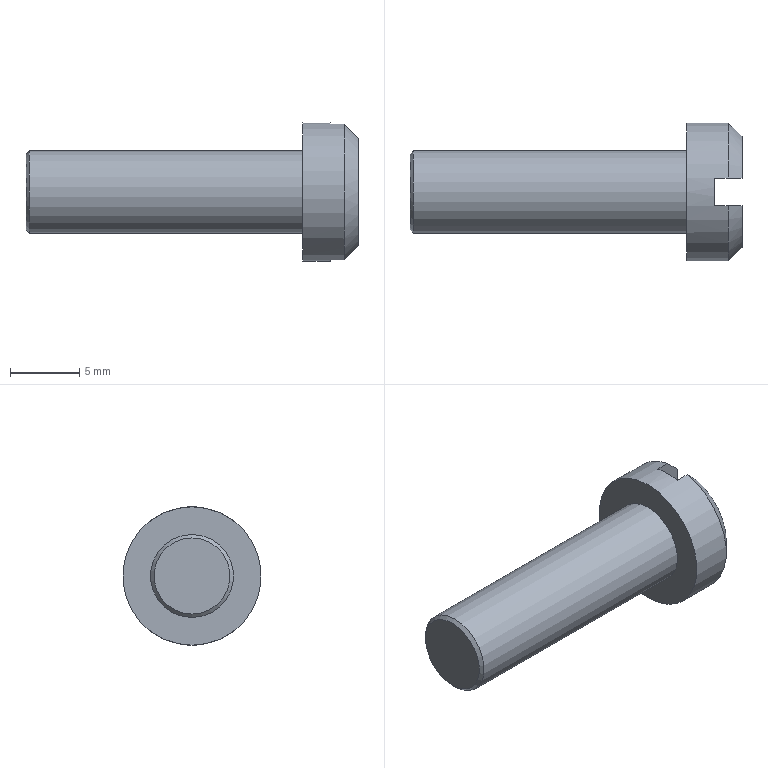Component | NX | SCREW2_2 | 1 solid | 12 faces | box 24 x 10 x 10 mm | volume 827 mm3 | plane 7 | cone 3 | cylinder 2 | commonest cylinder face diameters 10 x1 6 x1
STEP:
#1=CARTESIAN_POINT('',(0.,0.,0.));
#2=DIRECTION('',(0.,0.,1.));
#3=DIRECTION('',(1.,0.,0.));
#4=AXIS2_PLACEMENT_3D('',#1,#2,#3);
#5=CARTESIAN_POINT('',(54.,39.,45.627));
#6=VERTEX_POINT('',#5);
#7=CARTESIAN_POINT('',(54.,39.,53.373));
#8=VERTEX_POINT('',#7);
#9=CARTESIAN_POINT('',(54.,39.,42.282));
#10=DIRECTION('',(0.,0.,1.));
#11=VECTOR('',#10,1.);
#12=LINE('',#9,#11);
#13=CARTESIAN_POINT('',(54.,40.,49.5));
#14=DIRECTION('',(1.,0.,0.));
#15=DIRECTION('',(0.,0.,-1.));
#16=AXIS2_PLACEMENT_3D('',#13,#14,#15);
#17=PLANE('',#16);
#18=CARTESIAN_POINT('',(7.218,-1.));
#19=DIRECTION('',(-1.,0.));
#20=VECTOR('',#19,1.);
#21=LINE('',#18,#20);
#22=(GEOMETRIC_REPRESENTATION_CONTEXT(2)PARAMETRIC_REPRESENTATION_CONTEXT()REPRESENTATION_CONTEXT('',''));
#23=DEFINITIONAL_REPRESENTATION('',(#21),#22);
#24=PCURVE('',#17,#23);
#25=CARTESIAN_POINT('',(52.,39.,42.282));
#26=DIRECTION('',(0.,1.,0.));
#27=DIRECTION('',(1.,0.,0.));
#28=AXIS2_PLACEMENT_3D('',#25,#26,#27);
#29=PLANE('',#28);
#30=CARTESIAN_POINT('',(2.,0.));
#31=DIRECTION('',(0.,-1.));
#32=VECTOR('',#31,1.);
#33=LINE('',#30,#32);
#34=(GEOMETRIC_REPRESENTATION_CONTEXT(2)PARAMETRIC_REPRESENTATION_CONTEXT()REPRESENTATION_CONTEXT('',''));
#35=DEFINITIONAL_REPRESENTATION('',(#33),#34);
#36=PCURVE('',#29,#35);
#37=SURFACE_CURVE('',#12,(#24,#36),.PCURVE_S1.);
#38=EDGE_CURVE('',#6,#8,#37,.T.);
#39=ORIENTED_EDGE('',*,*,#38,.T.);
#40=CARTESIAN_POINT('',(54.,40.,49.5));
#41=DIRECTION('',(1.,0.,0.));
#42=DIRECTION('',(0.,0.,-1.));
#43=AXIS2_PLACEMENT_3D('',#40,#41,#42);
#44=CIRCLE('',#43,4.);
#45=CARTESIAN_POINT('',(0.,0.));
#46=DIRECTION('',(1.,0.));
#47=AXIS2_PLACEMENT_2D('',#45,#46);
#48=CIRCLE('',#47,4.);
#49=(GEOMETRIC_REPRESENTATION_CONTEXT(2)PARAMETRIC_REPRESENTATION_CONTEXT()REPRESENTATION_CONTEXT('',''));
#50=DEFINITIONAL_REPRESENTATION('',(#48),#49);
#51=PCURVE('',#17,#50);
#52=CARTESIAN_POINT('',(54.,40.,49.5));
#53=DIRECTION('',(-1.,0.,0.));
#54=DIRECTION('',(0.,0.,1.));
#55=AXIS2_PLACEMENT_3D('',#52,#53,#54);
#56=CONICAL_SURFACE('',#55,4.,0.7854);
#57=CARTESIAN_POINT('',(9.425,0.));
#58=DIRECTION('',(-1.,-0.));
#59=VECTOR('',#58,1.);
#60=LINE('',#57,#59);
#61=(GEOMETRIC_REPRESENTATION_CONTEXT(2)PARAMETRIC_REPRESENTATION_CONTEXT()REPRESENTATION_CONTEXT('',''));
#62=DEFINITIONAL_REPRESENTATION('',(#60),#61);
#63=PCURVE('',#56,#62);
#64=SURFACE_CURVE('',#44,(#51,#63),.PCURVE_S1.);
#65=EDGE_CURVE('',#8,#6,#64,.T.);
#66=ORIENTED_EDGE('',*,*,#65,.T.);
#67=EDGE_LOOP('',(#39,#66));
#68=FACE_BOUND('',#67,.T.);
#69=ADVANCED_FACE('',(#68),#17,.T.);
#70=CARTESIAN_POINT('',(54.,41.,53.373));
#71=VERTEX_POINT('',#70);
#72=CARTESIAN_POINT('',(54.,41.,45.627));
#73=VERTEX_POINT('',#72);
#74=CARTESIAN_POINT('',(54.,41.,56.718));
#75=DIRECTION('',(0.,0.,-1.));
#76=VECTOR('',#75,1.);
#77=LINE('',#74,#76);
#78=CARTESIAN_POINT('',(54.,40.,49.5));
#79=DIRECTION('',(1.,0.,0.));
#80=DIRECTION('',(0.,0.,-1.));
#81=AXIS2_PLACEMENT_3D('',#78,#79,#80);
#82=PLANE('',#81);
#83=CARTESIAN_POINT('',(-7.218,1.));
#84=DIRECTION('',(1.,0.));
#85=VECTOR('',#84,1.);
#86=LINE('',#83,#85);
#87=(GEOMETRIC_REPRESENTATION_CONTEXT(2)PARAMETRIC_REPRESENTATION_CONTEXT()REPRESENTATION_CONTEXT('',''));
#88=DEFINITIONAL_REPRESENTATION('',(#86),#87);
#89=PCURVE('',#82,#88);
#90=CARTESIAN_POINT('',(52.,41.,56.718));
#91=DIRECTION('',(0.,-1.,0.));
#92=DIRECTION('',(-1.,0.,0.));
#93=AXIS2_PLACEMENT_3D('',#90,#91,#92);
#94=PLANE('',#93);
#95=CARTESIAN_POINT('',(-2.,0.));
#96=DIRECTION('',(0.,1.));
#97=VECTOR('',#96,1.);
#98=LINE('',#95,#97);
#99=(GEOMETRIC_REPRESENTATION_CONTEXT(2)PARAMETRIC_REPRESENTATION_CONTEXT()REPRESENTATION_CONTEXT('',''));
#100=DEFINITIONAL_REPRESENTATION('',(#98),#99);
#101=PCURVE('',#94,#100);
#102=SURFACE_CURVE('',#77,(#89,#101),.PCURVE_S1.);
#103=EDGE_CURVE('',#71,#73,#102,.T.);
#104=ORIENTED_EDGE('',*,*,#103,.T.);
#105=CARTESIAN_POINT('',(54.,40.,49.5));
#106=DIRECTION('',(1.,0.,0.));
#107=DIRECTION('',(0.,0.,-1.));
#108=AXIS2_PLACEMENT_3D('',#105,#106,#107);
#109=CIRCLE('',#108,4.);
#110=CARTESIAN_POINT('',(0.,0.));
#111=DIRECTION('',(1.,0.));
#112=AXIS2_PLACEMENT_2D('',#110,#111);
#113=CIRCLE('',#112,4.);
#114=(GEOMETRIC_REPRESENTATION_CONTEXT(2)PARAMETRIC_REPRESENTATION_CONTEXT()REPRESENTATION_CONTEXT('',''));
#115=DEFINITIONAL_REPRESENTATION('',(#113),#114);
#116=PCURVE('',#82,#115);
#117=CARTESIAN_POINT('',(54.,40.,49.5));
#118=DIRECTION('',(-1.,0.,0.));
#119=DIRECTION('',(0.,0.,1.));
#120=AXIS2_PLACEMENT_3D('',#117,#118,#119);
#121=CONICAL_SURFACE('',#120,4.,0.7854);
#122=CARTESIAN_POINT('',(3.142,0.));
#123=DIRECTION('',(-1.,0.));
#124=VECTOR('',#123,1.);
#125=LINE('',#122,#124);
#126=(GEOMETRIC_REPRESENTATION_CONTEXT(2)PARAMETRIC_REPRESENTATION_CONTEXT()REPRESENTATION_CONTEXT('',''));
#127=DEFINITIONAL_REPRESENTATION('',(#125),#126);
#128=PCURVE('',#121,#127);
#129=SURFACE_CURVE('',#109,(#116,#128),.PCURVE_S1.);
#130=EDGE_CURVE('',#73,#71,#129,.T.);
#131=ORIENTED_EDGE('',*,*,#130,.T.);
#132=EDGE_LOOP('',(#104,#131));
#133=FACE_BOUND('',#132,.T.);
#134=ADVANCED_FACE('',(#133),#82,.T.);
#135=CARTESIAN_POINT('',(50.,40.,44.5));
#136=VERTEX_POINT('',#135);
#137=CARTESIAN_POINT('',(50.,40.,49.5));
#138=DIRECTION('',(1.,0.,0.));
#139=DIRECTION('',(0.,0.,-1.));
#140=AXIS2_PLACEMENT_3D('',#137,#138,#139);
#141=CIRCLE('',#140,5.);
#142=CARTESIAN_POINT('',(50.,40.,49.5));
#143=DIRECTION('',(1.,0.,0.));
#144=DIRECTION('',(0.,0.,-1.));
#145=AXIS2_PLACEMENT_3D('',#142,#143,#144);
#146=CYLINDRICAL_SURFACE('',#145,5.);
#147=CARTESIAN_POINT('',(0.,0.));
#148=DIRECTION('',(1.,0.));
#149=VECTOR('',#148,1.);
#150=LINE('',#147,#149);
#151=(GEOMETRIC_REPRESENTATION_CONTEXT(2)PARAMETRIC_REPRESENTATION_CONTEXT()REPRESENTATION_CONTEXT('',''));
#152=DEFINITIONAL_REPRESENTATION('',(#150),#151);
#153=PCURVE('',#146,#152);
#154=CARTESIAN_POINT('',(50.,40.,49.5));
#155=DIRECTION('',(-1.,0.,0.));
#156=DIRECTION('',(0.,0.,1.));
#157=AXIS2_PLACEMENT_3D('',#154,#155,#156);
#158=PLANE('',#157);
#159=CARTESIAN_POINT('',(-5.,0.));
#160=CARTESIAN_POINT('',(-5.,8.66));
#161=CARTESIAN_POINT('',(2.5,4.33));
#162=CARTESIAN_POINT('',(10.,0.));
#163=CARTESIAN_POINT('',(2.5,-4.33));
#164=CARTESIAN_POINT('',(-5.,-8.66));
#165=CARTESIAN_POINT('',(-5.,0.));
#166=(BOUNDED_CURVE()B_SPLINE_CURVE(2,(#159,#160,#161,#162,#163,#164,#165),.UNSPECIFIED.,.T.,.F.)B_SPLINE_CURVE_WITH_KNOTS((1,2,2,2,2,1),(-2.094,0.,2.094,4.189,6.283,8.378),.UNSPECIFIED.)CURVE()GEOMETRIC_REPRESENTATION_ITEM()RATIONAL_B_SPLINE_CURVE((1.,0.5,1.,0.5,1.,0.5,1.))REPRESENTATION_ITEM(''));
#167=(GEOMETRIC_REPRESENTATION_CONTEXT(2)PARAMETRIC_REPRESENTATION_CONTEXT()REPRESENTATION_CONTEXT('',''));
#168=DEFINITIONAL_REPRESENTATION('',(#166),#167);
#169=PCURVE('',#158,#168);
#170=SURFACE_CURVE('',#141,(#153,#169),.PCURVE_S1.);
#171=EDGE_CURVE('',#136,#136,#170,.T.);
#172=ORIENTED_EDGE('',*,*,#171,.T.);
#173=CARTESIAN_POINT('',(52.,40.,44.5));
#174=VERTEX_POINT('',#173);
#175=CARTESIAN_POINT('',(50.,40.,44.5));
#176=CARTESIAN_POINT('',(52.,40.,44.5));
#177=B_SPLINE_CURVE_WITH_KNOTS('',1,(#175,#176),.UNSPECIFIED.,.F.,.F.,(2,2),(0.,2.),.PIECEWISE_BEZIER_KNOTS.);
#178=CARTESIAN_POINT('',(6.283,0.));
#179=DIRECTION('',(0.,1.));
#180=VECTOR('',#179,1.);
#181=LINE('',#178,#180);
#182=(GEOMETRIC_REPRESENTATION_CONTEXT(2)PARAMETRIC_REPRESENTATION_CONTEXT()REPRESENTATION_CONTEXT('',''));
#183=DEFINITIONAL_REPRESENTATION('',(#181),#182);
#184=PCURVE('',#146,#183);
#185=CARTESIAN_POINT('',(0.,0.));
#186=DIRECTION('',(0.,1.));
#187=VECTOR('',#186,1.);
#188=LINE('',#185,#187);
#189=(GEOMETRIC_REPRESENTATION_CONTEXT(2)PARAMETRIC_REPRESENTATION_CONTEXT()REPRESENTATION_CONTEXT('',''));
#190=DEFINITIONAL_REPRESENTATION('',(#188),#189);
#191=PCURVE('',#146,#190);
#192=SEAM_CURVE('',#177,(#184,#191),.PCURVE_S1.);
#193=EDGE_CURVE('',#136,#174,#192,.T.);
#194=ORIENTED_EDGE('',*,*,#193,.T.);
#195=CARTESIAN_POINT('',(52.,39.,44.601));
#196=VERTEX_POINT('',#195);
#197=CARTESIAN_POINT('',(52.,40.,49.5));
#198=DIRECTION('',(1.,0.,0.));
#199=DIRECTION('',(0.,0.,1.));
#200=AXIS2_PLACEMENT_3D('',#197,#198,#199);
#201=CIRCLE('',#200,5.);
#202=CARTESIAN_POINT('',(3.142,2.));
#203=DIRECTION('',(1.,0.));
#204=VECTOR('',#203,1.);
#205=LINE('',#202,#204);
#206=(GEOMETRIC_REPRESENTATION_CONTEXT(2)PARAMETRIC_REPRESENTATION_CONTEXT()REPRESENTATION_CONTEXT('',''));
#207=DEFINITIONAL_REPRESENTATION('',(#205),#206);
#208=PCURVE('',#146,#207);
#209=CARTESIAN_POINT('',(52.,40.,49.5));
#210=DIRECTION('',(-1.,0.,0.));
#211=DIRECTION('',(0.,0.,1.));
#212=AXIS2_PLACEMENT_3D('',#209,#210,#211);
#213=PLANE('',#212);
#214=CARTESIAN_POINT('',(5.,0.));
#215=CARTESIAN_POINT('',(5.,-8.66));
#216=CARTESIAN_POINT('',(-2.5,-4.33));
#217=CARTESIAN_POINT('',(-10.,-0.));
#218=CARTESIAN_POINT('',(-2.5,4.33));
#219=CARTESIAN_POINT('',(5.,8.66));
#220=CARTESIAN_POINT('',(5.,0.));
#221=(BOUNDED_CURVE()B_SPLINE_CURVE(2,(#214,#215,#216,#217,#218,#219,#220),.UNSPECIFIED.,.T.,.F.)B_SPLINE_CURVE_WITH_KNOTS((1,2,2,2,2,1),(-2.094,0.,2.094,4.189,6.283,8.378),.UNSPECIFIED.)CURVE()GEOMETRIC_REPRESENTATION_ITEM()RATIONAL_B_SPLINE_CURVE((1.,0.5,1.,0.5,1.,0.5,1.))REPRESENTATION_ITEM(''));
#222=(GEOMETRIC_REPRESENTATION_CONTEXT(2)PARAMETRIC_REPRESENTATION_CONTEXT()REPRESENTATION_CONTEXT('',''));
#223=DEFINITIONAL_REPRESENTATION('',(#221),#222);
#224=PCURVE('',#213,#223);
#225=SURFACE_CURVE('',#201,(#208,#224),.PCURVE_S1.);
#226=EDGE_CURVE('',#196,#174,#225,.T.);
#227=ORIENTED_EDGE('',*,*,#226,.F.);
#228=CARTESIAN_POINT('',(53.,39.,44.601));
#229=VERTEX_POINT('',#228);
#230=CARTESIAN_POINT('',(50.,39.,44.601));
#231=DIRECTION('',(1.,0.,0.));
#232=VECTOR('',#231,1.);
#233=LINE('',#230,#232);
#234=CARTESIAN_POINT('',(6.082,0.));
#235=DIRECTION('',(0.,1.));
#236=VECTOR('',#235,1.);
#237=LINE('',#234,#236);
#238=(GEOMETRIC_REPRESENTATION_CONTEXT(2)PARAMETRIC_REPRESENTATION_CONTEXT()REPRESENTATION_CONTEXT('',''));
#239=DEFINITIONAL_REPRESENTATION('',(#237),#238);
#240=PCURVE('',#146,#239);
#241=CARTESIAN_POINT('',(-2.,-2.319));
#242=DIRECTION('',(1.,0.));
#243=VECTOR('',#242,1.);
#244=LINE('',#241,#243);
#245=(GEOMETRIC_REPRESENTATION_CONTEXT(2)PARAMETRIC_REPRESENTATION_CONTEXT()REPRESENTATION_CONTEXT('',''));
#246=DEFINITIONAL_REPRESENTATION('',(#244),#245);
#247=PCURVE('',#29,#246);
#248=SURFACE_CURVE('',#233,(#240,#247),.PCURVE_S1.);
#249=EDGE_CURVE('',#196,#229,#248,.T.);
#250=ORIENTED_EDGE('',*,*,#249,.T.);
#251=CARTESIAN_POINT('',(53.,39.,54.399));
#252=VERTEX_POINT('',#251);
#253=CARTESIAN_POINT('',(53.,40.,49.5));
#254=DIRECTION('',(-1.,0.,0.));
#255=DIRECTION('',(0.,0.,-1.));
#256=AXIS2_PLACEMENT_3D('',#253,#254,#255);
#257=CIRCLE('',#256,5.);
#258=CARTESIAN_POINT('',(6.283,3.));
#259=DIRECTION('',(-1.,0.));
#260=VECTOR('',#259,1.);
#261=LINE('',#258,#260);
#262=(GEOMETRIC_REPRESENTATION_CONTEXT(2)PARAMETRIC_REPRESENTATION_CONTEXT()REPRESENTATION_CONTEXT('',''));
#263=DEFINITIONAL_REPRESENTATION('',(#261),#262);
#264=PCURVE('',#146,#263);
#265=CARTESIAN_POINT('',(3.142,1.));
#266=DIRECTION('',(1.,0.));
#267=VECTOR('',#266,1.);
#268=LINE('',#265,#267);
#269=(GEOMETRIC_REPRESENTATION_CONTEXT(2)PARAMETRIC_REPRESENTATION_CONTEXT()REPRESENTATION_CONTEXT('',''));
#270=DEFINITIONAL_REPRESENTATION('',(#268),#269);
#271=PCURVE('',#56,#270);
#272=SURFACE_CURVE('',#257,(#264,#271),.PCURVE_S1.);
#273=EDGE_CURVE('',#229,#252,#272,.T.);
#274=ORIENTED_EDGE('',*,*,#273,.T.);
#275=CARTESIAN_POINT('',(52.,39.,54.399));
#276=VERTEX_POINT('',#275);
#277=CARTESIAN_POINT('',(50.,39.,54.399));
#278=DIRECTION('',(-1.,0.,0.));
#279=VECTOR('',#278,1.);
#280=LINE('',#277,#279);
#281=CARTESIAN_POINT('',(3.343,0.));
#282=DIRECTION('',(0.,-1.));
#283=VECTOR('',#282,1.);
#284=LINE('',#281,#283);
#285=(GEOMETRIC_REPRESENTATION_CONTEXT(2)PARAMETRIC_REPRESENTATION_CONTEXT()REPRESENTATION_CONTEXT('',''));
#286=DEFINITIONAL_REPRESENTATION('',(#284),#285);
#287=PCURVE('',#146,#286);
#288=CARTESIAN_POINT('',(-2.,-12.116));
#289=DIRECTION('',(-1.,0.));
#290=VECTOR('',#289,1.);
#291=LINE('',#288,#290);
#292=(GEOMETRIC_REPRESENTATION_CONTEXT(2)PARAMETRIC_REPRESENTATION_CONTEXT()REPRESENTATION_CONTEXT('',''));
#293=DEFINITIONAL_REPRESENTATION('',(#291),#292);
#294=PCURVE('',#29,#293);
#295=SURFACE_CURVE('',#280,(#287,#294),.PCURVE_S1.);
#296=EDGE_CURVE('',#252,#276,#295,.T.);
#297=ORIENTED_EDGE('',*,*,#296,.T.);
#298=CARTESIAN_POINT('',(52.,41.,54.399));
#299=VERTEX_POINT('',#298);
#300=CARTESIAN_POINT('',(52.,40.,49.5));
#301=DIRECTION('',(1.,0.,0.));
#302=DIRECTION('',(0.,0.,1.));
#303=AXIS2_PLACEMENT_3D('',#300,#301,#302);
#304=CIRCLE('',#303,5.);
#305=CARTESIAN_POINT('',(-3.142,2.));
#306=DIRECTION('',(1.,0.));
#307=VECTOR('',#306,1.);
#308=LINE('',#305,#307);
#309=(GEOMETRIC_REPRESENTATION_CONTEXT(2)PARAMETRIC_REPRESENTATION_CONTEXT()REPRESENTATION_CONTEXT('',''));
#310=DEFINITIONAL_REPRESENTATION('',(#308),#309);
#311=PCURVE('',#146,#310);
#312=CARTESIAN_POINT('',(5.,0.));
#313=CARTESIAN_POINT('',(5.,-8.66));
#314=CARTESIAN_POINT('',(-2.5,-4.33));
#315=CARTESIAN_POINT('',(-10.,-0.));
#316=CARTESIAN_POINT('',(-2.5,4.33));
#317=CARTESIAN_POINT('',(5.,8.66));
#318=CARTESIAN_POINT('',(5.,0.));
#319=(BOUNDED_CURVE()B_SPLINE_CURVE(2,(#312,#313,#314,#315,#316,#317,#318),.UNSPECIFIED.,.T.,.F.)B_SPLINE_CURVE_WITH_KNOTS((1,2,2,2,2,1),(-2.094,0.,2.094,4.189,6.283,8.378),.UNSPECIFIED.)CURVE()GEOMETRIC_REPRESENTATION_ITEM()RATIONAL_B_SPLINE_CURVE((1.,0.5,1.,0.5,1.,0.5,1.))REPRESENTATION_ITEM(''));
#320=(GEOMETRIC_REPRESENTATION_CONTEXT(2)PARAMETRIC_REPRESENTATION_CONTEXT()REPRESENTATION_CONTEXT('',''));
#321=DEFINITIONAL_REPRESENTATION('',(#319),#320);
#322=PCURVE('',#213,#321);
#323=SURFACE_CURVE('',#304,(#311,#322),.PCURVE_S1.);
#324=EDGE_CURVE('',#299,#276,#323,.T.);
#325=ORIENTED_EDGE('',*,*,#324,.F.);
#326=CARTESIAN_POINT('',(53.,41.,54.399));
#327=VERTEX_POINT('',#326);
#328=CARTESIAN_POINT('',(50.,41.,54.399));
#329=DIRECTION('',(1.,0.,0.));
#330=VECTOR('',#329,1.);
#331=LINE('',#328,#330);
#332=CARTESIAN_POINT('',(2.94,0.));
#333=DIRECTION('',(0.,1.));
#334=VECTOR('',#333,1.);
#335=LINE('',#332,#334);
#336=(GEOMETRIC_REPRESENTATION_CONTEXT(2)PARAMETRIC_REPRESENTATION_CONTEXT()REPRESENTATION_CONTEXT('',''));
#337=DEFINITIONAL_REPRESENTATION('',(#335),#336);
#338=PCURVE('',#146,#337);
#339=CARTESIAN_POINT('',(2.,2.319));
#340=DIRECTION('',(-1.,0.));
#341=VECTOR('',#340,1.);
#342=LINE('',#339,#341);
#343=(GEOMETRIC_REPRESENTATION_CONTEXT(2)PARAMETRIC_REPRESENTATION_CONTEXT()REPRESENTATION_CONTEXT('',''));
#344=DEFINITIONAL_REPRESENTATION('',(#342),#343);
#345=PCURVE('',#94,#344);
#346=SURFACE_CURVE('',#331,(#338,#345),.PCURVE_S1.);
#347=EDGE_CURVE('',#299,#327,#346,.T.);
#348=ORIENTED_EDGE('',*,*,#347,.T.);
#349=CARTESIAN_POINT('',(53.,41.,44.601));
#350=VERTEX_POINT('',#349);
#351=CARTESIAN_POINT('',(53.,40.,49.5));
#352=DIRECTION('',(-1.,0.,0.));
#353=DIRECTION('',(0.,0.,-1.));
#354=AXIS2_PLACEMENT_3D('',#351,#352,#353);
#355=CIRCLE('',#354,5.);
#356=CARTESIAN_POINT('',(6.283,3.));
#357=DIRECTION('',(-1.,0.));
#358=VECTOR('',#357,1.);
#359=LINE('',#356,#358);
#360=(GEOMETRIC_REPRESENTATION_CONTEXT(2)PARAMETRIC_REPRESENTATION_CONTEXT()REPRESENTATION_CONTEXT('',''));
#361=DEFINITIONAL_REPRESENTATION('',(#359),#360);
#362=PCURVE('',#146,#361);
#363=CARTESIAN_POINT('',(-3.142,1.));
#364=DIRECTION('',(1.,0.));
#365=VECTOR('',#364,1.);
#366=LINE('',#363,#365);
#367=(GEOMETRIC_REPRESENTATION_CONTEXT(2)PARAMETRIC_REPRESENTATION_CONTEXT()REPRESENTATION_CONTEXT('',''));
#368=DEFINITIONAL_REPRESENTATION('',(#366),#367);
#369=PCURVE('',#121,#368);
#370=SURFACE_CURVE('',#355,(#362,#369),.PCURVE_S1.);
#371=EDGE_CURVE('',#327,#350,#370,.T.);
#372=ORIENTED_EDGE('',*,*,#371,.T.);
#373=CARTESIAN_POINT('',(52.,41.,44.601));
#374=VERTEX_POINT('',#373);
#375=CARTESIAN_POINT('',(50.,41.,44.601));
#376=DIRECTION('',(-1.,0.,0.));
#377=VECTOR('',#376,1.);
#378=LINE('',#375,#377);
#379=CARTESIAN_POINT('',(0.2014,0.));
#380=DIRECTION('',(0.,-1.));
#381=VECTOR('',#380,1.);
#382=LINE('',#379,#381);
#383=(GEOMETRIC_REPRESENTATION_CONTEXT(2)PARAMETRIC_REPRESENTATION_CONTEXT()REPRESENTATION_CONTEXT('',''));
#384=DEFINITIONAL_REPRESENTATION('',(#382),#383);
#385=PCURVE('',#146,#384);
#386=CARTESIAN_POINT('',(2.,12.116));
#387=DIRECTION('',(1.,0.));
#388=VECTOR('',#387,1.);
#389=LINE('',#386,#388);
#390=(GEOMETRIC_REPRESENTATION_CONTEXT(2)PARAMETRIC_REPRESENTATION_CONTEXT()REPRESENTATION_CONTEXT('',''));
#391=DEFINITIONAL_REPRESENTATION('',(#389),#390);
#392=PCURVE('',#94,#391);
#393=SURFACE_CURVE('',#378,(#385,#392),.PCURVE_S1.);
#394=EDGE_CURVE('',#350,#374,#393,.T.);
#395=ORIENTED_EDGE('',*,*,#394,.T.);
#396=CARTESIAN_POINT('',(52.,40.,49.5));
#397=DIRECTION('',(1.,0.,0.));
#398=DIRECTION('',(0.,0.,1.));
#399=AXIS2_PLACEMENT_3D('',#396,#397,#398);
#400=CIRCLE('',#399,5.);
#401=CARTESIAN_POINT('',(-3.142,2.));
#402=DIRECTION('',(1.,0.));
#403=VECTOR('',#402,1.);
#404=LINE('',#401,#403);
#405=(GEOMETRIC_REPRESENTATION_CONTEXT(2)PARAMETRIC_REPRESENTATION_CONTEXT()REPRESENTATION_CONTEXT('',''));
#406=DEFINITIONAL_REPRESENTATION('',(#404),#405);
#407=PCURVE('',#146,#406);
#408=CARTESIAN_POINT('',(5.,0.));
#409=CARTESIAN_POINT('',(5.,-8.66));
#410=CARTESIAN_POINT('',(-2.5,-4.33));
#411=CARTESIAN_POINT('',(-10.,-0.));
#412=CARTESIAN_POINT('',(-2.5,4.33));
#413=CARTESIAN_POINT('',(5.,8.66));
#414=CARTESIAN_POINT('',(5.,0.));
#415=(BOUNDED_CURVE()B_SPLINE_CURVE(2,(#408,#409,#410,#411,#412,#413,#414),.UNSPECIFIED.,.T.,.F.)B_SPLINE_CURVE_WITH_KNOTS((1,2,2,2,2,1),(-2.094,0.,2.094,4.189,6.283,8.378),.UNSPECIFIED.)CURVE()GEOMETRIC_REPRESENTATION_ITEM()RATIONAL_B_SPLINE_CURVE((1.,0.5,1.,0.5,1.,0.5,1.))REPRESENTATION_ITEM(''));
#416=(GEOMETRIC_REPRESENTATION_CONTEXT(2)PARAMETRIC_REPRESENTATION_CONTEXT()REPRESENTATION_CONTEXT('',''));
#417=DEFINITIONAL_REPRESENTATION('',(#415),#416);
#418=PCURVE('',#213,#417);
#419=SURFACE_CURVE('',#400,(#407,#418),.PCURVE_S1.);
#420=EDGE_CURVE('',#174,#374,#419,.T.);
#421=ORIENTED_EDGE('',*,*,#420,.F.);
#422=ORIENTED_EDGE('',*,*,#193,.F.);
#423=EDGE_LOOP('',(#172,#194,#227,#250,#274,#297,#325,#348,#372,#395,#421,#422));
#424=FACE_BOUND('',#423,.T.);
#425=ADVANCED_FACE('',(#424),#146,.T.);
#426=CARTESIAN_POINT('',(30.,40.,52.25));
#427=VERTEX_POINT('',#426);
#428=CARTESIAN_POINT('',(30.,40.,49.5));
#429=DIRECTION('',(-1.,0.,0.));
#430=DIRECTION('',(0.,0.,1.));
#431=AXIS2_PLACEMENT_3D('',#428,#429,#430);
#432=CIRCLE('',#431,2.75);
#433=CARTESIAN_POINT('',(30.,40.,49.5));
#434=DIRECTION('',(-1.,0.,0.));
#435=DIRECTION('',(0.,0.,1.));
#436=AXIS2_PLACEMENT_3D('',#433,#434,#435);
#437=PLANE('',#436);
#438=CARTESIAN_POINT('',(0.,0.));
#439=DIRECTION('',(1.,0.));
#440=AXIS2_PLACEMENT_2D('',#438,#439);
#441=CIRCLE('',#440,2.75);
#442=(GEOMETRIC_REPRESENTATION_CONTEXT(2)PARAMETRIC_REPRESENTATION_CONTEXT()REPRESENTATION_CONTEXT('',''));
#443=DEFINITIONAL_REPRESENTATION('',(#441),#442);
#444=PCURVE('',#437,#443);
#445=CARTESIAN_POINT('',(30.25,40.,49.5));
#446=DIRECTION('',(1.,0.,0.));
#447=DIRECTION('',(0.,0.,-1.));
#448=AXIS2_PLACEMENT_3D('',#445,#446,#447);
#449=CONICAL_SURFACE('',#448,3.,0.7854);
#450=CARTESIAN_POINT('',(9.425,-0.25));
#451=DIRECTION('',(-1.,0.));
#452=VECTOR('',#451,1.);
#453=LINE('',#450,#452);
#454=(GEOMETRIC_REPRESENTATION_CONTEXT(2)PARAMETRIC_REPRESENTATION_CONTEXT()REPRESENTATION_CONTEXT('',''));
#455=DEFINITIONAL_REPRESENTATION('',(#453),#454);
#456=PCURVE('',#449,#455);
#457=SURFACE_CURVE('',#432,(#444,#456),.PCURVE_S1.);
#458=EDGE_CURVE('',#427,#427,#457,.T.);
#459=ORIENTED_EDGE('',*,*,#458,.T.);
#460=EDGE_LOOP('',(#459));
#461=FACE_BOUND('',#460,.T.);
#462=ADVANCED_FACE('',(#461),#437,.T.);
#463=CARTESIAN_POINT('',(30.25,40.,52.5));
#464=VERTEX_POINT('',#463);
#465=CARTESIAN_POINT('',(30.25,40.,46.5));
#466=VERTEX_POINT('',#465);
#467=CARTESIAN_POINT('',(30.25,40.,49.5));
#468=DIRECTION('',(1.,0.,0.));
#469=DIRECTION('',(0.,0.,1.));
#470=AXIS2_PLACEMENT_3D('',#467,#468,#469);
#471=CIRCLE('',#470,3.);
#472=CARTESIAN_POINT('',(30.,40.,49.5));
#473=DIRECTION('',(1.,0.,0.));
#474=DIRECTION('',(0.,0.,-1.));
#475=AXIS2_PLACEMENT_3D('',#472,#473,#474);
#476=CYLINDRICAL_SURFACE('',#475,3.);
#477=CARTESIAN_POINT('',(3.142,0.25));
#478=DIRECTION('',(1.,0.));
#479=VECTOR('',#478,1.);
#480=LINE('',#477,#479);
#481=(GEOMETRIC_REPRESENTATION_CONTEXT(2)PARAMETRIC_REPRESENTATION_CONTEXT()REPRESENTATION_CONTEXT('',''));
#482=DEFINITIONAL_REPRESENTATION('',(#480),#481);
#483=PCURVE('',#476,#482);
#484=CARTESIAN_POINT('',(3.142,0.));
#485=DIRECTION('',(1.,0.));
#486=VECTOR('',#485,1.);
#487=LINE('',#484,#486);
#488=(GEOMETRIC_REPRESENTATION_CONTEXT(2)PARAMETRIC_REPRESENTATION_CONTEXT()REPRESENTATION_CONTEXT('',''));
#489=DEFINITIONAL_REPRESENTATION('',(#487),#488);
#490=PCURVE('',#449,#489);
#491=SURFACE_CURVE('',#471,(#483,#490),.PCURVE_S1.);
#492=EDGE_CURVE('',#464,#466,#491,.T.);
#493=ORIENTED_EDGE('',*,*,#492,.T.);
#494=CARTESIAN_POINT('',(50.,40.,46.5));
#495=VERTEX_POINT('',#494);
#496=CARTESIAN_POINT('',(30.25,40.,46.5));
#497=CARTESIAN_POINT('',(50.,40.,46.5));
#498=B_SPLINE_CURVE_WITH_KNOTS('',1,(#496,#497),.UNSPECIFIED.,.F.,.F.,(2,2),(0.25,20.),.PIECEWISE_BEZIER_KNOTS.);
#499=CARTESIAN_POINT('',(6.283,0.));
#500=DIRECTION('',(0.,1.));
#501=VECTOR('',#500,1.);
#502=LINE('',#499,#501);
#503=(GEOMETRIC_REPRESENTATION_CONTEXT(2)PARAMETRIC_REPRESENTATION_CONTEXT()REPRESENTATION_CONTEXT('',''));
#504=DEFINITIONAL_REPRESENTATION('',(#502),#503);
#505=PCURVE('',#476,#504);
#506=CARTESIAN_POINT('',(0.,0.));
#507=DIRECTION('',(0.,1.));
#508=VECTOR('',#507,1.);
#509=LINE('',#506,#508);
#510=(GEOMETRIC_REPRESENTATION_CONTEXT(2)PARAMETRIC_REPRESENTATION_CONTEXT()REPRESENTATION_CONTEXT('',''));
#511=DEFINITIONAL_REPRESENTATION('',(#509),#510);
#512=PCURVE('',#476,#511);
#513=SEAM_CURVE('',#498,(#505,#512),.PCURVE_S1.);
#514=EDGE_CURVE('',#466,#495,#513,.T.);
#515=ORIENTED_EDGE('',*,*,#514,.T.);
#516=CARTESIAN_POINT('',(50.,40.,49.5));
#517=DIRECTION('',(-1.,0.,0.));
#518=DIRECTION('',(0.,0.,-1.));
#519=AXIS2_PLACEMENT_3D('',#516,#517,#518);
#520=CIRCLE('',#519,3.);
#521=CARTESIAN_POINT('',(6.283,20.));
#522=DIRECTION('',(-1.,0.));
#523=VECTOR('',#522,1.);
#524=LINE('',#521,#523);
#525=(GEOMETRIC_REPRESENTATION_CONTEXT(2)PARAMETRIC_REPRESENTATION_CONTEXT()REPRESENTATION_CONTEXT('',''));
#526=DEFINITIONAL_REPRESENTATION('',(#524),#525);
#527=PCURVE('',#476,#526);
#528=CARTESIAN_POINT('',(0.,0.));
#529=DIRECTION('',(-1.,0.));
#530=AXIS2_PLACEMENT_2D('',#528,#529);
#531=CIRCLE('',#530,3.);
#532=(GEOMETRIC_REPRESENTATION_CONTEXT(2)PARAMETRIC_REPRESENTATION_CONTEXT()REPRESENTATION_CONTEXT('',''));
#533=DEFINITIONAL_REPRESENTATION('',(#531),#532);
#534=PCURVE('',#158,#533);
#535=SURFACE_CURVE('',#520,(#527,#534),.PCURVE_S1.);
#536=EDGE_CURVE('',#495,#495,#535,.T.);
#537=ORIENTED_EDGE('',*,*,#536,.T.);
#538=ORIENTED_EDGE('',*,*,#514,.F.);
#539=CARTESIAN_POINT('',(30.25,40.,49.5));
#540=DIRECTION('',(1.,0.,0.));
#541=DIRECTION('',(0.,0.,1.));
#542=AXIS2_PLACEMENT_3D('',#539,#540,#541);
#543=CIRCLE('',#542,3.);
#544=CARTESIAN_POINT('',(-3.142,0.25));
#545=DIRECTION('',(1.,0.));
#546=VECTOR('',#545,1.);
#547=LINE('',#544,#546);
#548=(GEOMETRIC_REPRESENTATION_CONTEXT(2)PARAMETRIC_REPRESENTATION_CONTEXT()REPRESENTATION_CONTEXT('',''));
#549=DEFINITIONAL_REPRESENTATION('',(#547),#548);
#550=PCURVE('',#476,#549);
#551=CARTESIAN_POINT('',(3.142,0.));
#552=DIRECTION('',(1.,0.));
#553=VECTOR('',#552,1.);
#554=LINE('',#551,#553);
#555=(GEOMETRIC_REPRESENTATION_CONTEXT(2)PARAMETRIC_REPRESENTATION_CONTEXT()REPRESENTATION_CONTEXT('',''));
#556=DEFINITIONAL_REPRESENTATION('',(#554),#555);
#557=PCURVE('',#449,#556);
#558=SURFACE_CURVE('',#543,(#550,#557),.PCURVE_S1.);
#559=EDGE_CURVE('',#466,#464,#558,.T.);
#560=ORIENTED_EDGE('',*,*,#559,.T.);
#561=EDGE_LOOP('',(#493,#515,#537,#538,#560));
#562=FACE_BOUND('',#561,.T.);
#563=ADVANCED_FACE('',(#562),#476,.T.);
#564=ORIENTED_EDGE('',*,*,#536,.F.);
#565=EDGE_LOOP('',(#564));
#566=FACE_BOUND('',#565,.T.);
#567=ORIENTED_EDGE('',*,*,#171,.F.);
#568=EDGE_LOOP('',(#567));
#569=FACE_BOUND('',#568,.T.);
#570=ADVANCED_FACE('',(#566,#569),#158,.T.);
#571=ORIENTED_EDGE('',*,*,#458,.F.);
#572=CARTESIAN_POINT('',(30.,40.,52.25));
#573=CARTESIAN_POINT('',(30.25,40.,52.5));
#574=B_SPLINE_CURVE_WITH_KNOTS('',1,(#572,#573),.UNSPECIFIED.,.F.,.F.,(2,2),(-0.3536,0.),.PIECEWISE_BEZIER_KNOTS.);
#575=CARTESIAN_POINT('',(9.425,0.));
#576=DIRECTION('',(0.,1.));
#577=VECTOR('',#576,1.);
#578=LINE('',#575,#577);
#579=(GEOMETRIC_REPRESENTATION_CONTEXT(2)PARAMETRIC_REPRESENTATION_CONTEXT()REPRESENTATION_CONTEXT('',''));
#580=DEFINITIONAL_REPRESENTATION('',(#578),#579);
#581=PCURVE('',#449,#580);
#582=CARTESIAN_POINT('',(3.142,0.));
#583=DIRECTION('',(0.,1.));
#584=VECTOR('',#583,1.);
#585=LINE('',#582,#584);
#586=(GEOMETRIC_REPRESENTATION_CONTEXT(2)PARAMETRIC_REPRESENTATION_CONTEXT()REPRESENTATION_CONTEXT('',''));
#587=DEFINITIONAL_REPRESENTATION('',(#585),#586);
#588=PCURVE('',#449,#587);
#589=SEAM_CURVE('',#574,(#581,#588),.PCURVE_S1.);
#590=EDGE_CURVE('',#427,#464,#589,.T.);
#591=ORIENTED_EDGE('',*,*,#590,.T.);
#592=ORIENTED_EDGE('',*,*,#559,.F.);
#593=ORIENTED_EDGE('',*,*,#492,.F.);
#594=ORIENTED_EDGE('',*,*,#590,.F.);
#595=EDGE_LOOP('',(#571,#591,#592,#593,#594));
#596=FACE_BOUND('',#595,.T.);
#597=ADVANCED_FACE('',(#596),#449,.T.);
#598=ORIENTED_EDGE('',*,*,#38,.F.);
#599=CARTESIAN_POINT('',(54.,39.,45.627));
#600=CARTESIAN_POINT('',(53.668,39.,45.284));
#601=CARTESIAN_POINT('',(53.334,39.,44.942));
#602=CARTESIAN_POINT('',(53.,39.,44.601));
#603=B_SPLINE_CURVE_WITH_KNOTS('',3,(#599,#600,#601,#602),.UNSPECIFIED.,.F.,.F.,(4,4),(0.,1.),.PIECEWISE_BEZIER_KNOTS.);
#604=CARTESIAN_POINT('',(2.,-3.345));
#605=CARTESIAN_POINT('',(1.668,-3.001));
#606=CARTESIAN_POINT('',(1.334,-2.66));
#607=CARTESIAN_POINT('',(1.,-2.319));
#608=B_SPLINE_CURVE_WITH_KNOTS('',3,(#604,#605,#606,#607),.UNSPECIFIED.,.F.,.F.,(4,4),(0.,1.),.PIECEWISE_BEZIER_KNOTS.);
#609=(GEOMETRIC_REPRESENTATION_CONTEXT(2)PARAMETRIC_REPRESENTATION_CONTEXT()REPRESENTATION_CONTEXT('',''));
#610=DEFINITIONAL_REPRESENTATION('',(#608),#609);
#611=PCURVE('',#29,#610);
#612=CARTESIAN_POINT('',(3.394,-0.));
#613=CARTESIAN_POINT('',(3.343,1.));
#614=B_SPLINE_CURVE_WITH_KNOTS('',1,(#612,#613),.UNSPECIFIED.,.F.,.F.,(2,2),(0.,1.),.PIECEWISE_BEZIER_KNOTS.);
#615=(GEOMETRIC_REPRESENTATION_CONTEXT(2)PARAMETRIC_REPRESENTATION_CONTEXT()REPRESENTATION_CONTEXT('',''));
#616=DEFINITIONAL_REPRESENTATION('',(#614),#615);
#617=PCURVE('',#56,#616);
#618=SURFACE_CURVE('',#603,(#611,#617),.PCURVE_S1.);
#619=EDGE_CURVE('',#6,#229,#618,.T.);
#620=ORIENTED_EDGE('',*,*,#619,.T.);
#621=ORIENTED_EDGE('',*,*,#249,.F.);
#622=CARTESIAN_POINT('',(52.,39.,42.282));
#623=DIRECTION('',(0.,0.,-1.));
#624=VECTOR('',#623,1.);
#625=LINE('',#622,#624);
#626=CARTESIAN_POINT('',(0.,0.));
#627=DIRECTION('',(0.,1.));
#628=VECTOR('',#627,1.);
#629=LINE('',#626,#628);
#630=(GEOMETRIC_REPRESENTATION_CONTEXT(2)PARAMETRIC_REPRESENTATION_CONTEXT()REPRESENTATION_CONTEXT('',''));
#631=DEFINITIONAL_REPRESENTATION('',(#629),#630);
#632=PCURVE('',#29,#631);
#633=CARTESIAN_POINT('',(-7.218,-1.));
#634=DIRECTION('',(-1.,0.));
#635=VECTOR('',#634,1.);
#636=LINE('',#633,#635);
#637=(GEOMETRIC_REPRESENTATION_CONTEXT(2)PARAMETRIC_REPRESENTATION_CONTEXT()REPRESENTATION_CONTEXT('',''));
#638=DEFINITIONAL_REPRESENTATION('',(#636),#637);
#639=PCURVE('',#213,#638);
#640=SURFACE_CURVE('',#625,(#632,#639),.PCURVE_S1.);
#641=EDGE_CURVE('',#276,#196,#640,.T.);
#642=ORIENTED_EDGE('',*,*,#641,.F.);
#643=ORIENTED_EDGE('',*,*,#296,.F.);
#644=CARTESIAN_POINT('',(53.,39.,54.399));
#645=CARTESIAN_POINT('',(53.334,39.,54.058));
#646=CARTESIAN_POINT('',(53.668,39.,53.716));
#647=CARTESIAN_POINT('',(54.,39.,53.373));
#648=B_SPLINE_CURVE_WITH_KNOTS('',3,(#644,#645,#646,#647),.UNSPECIFIED.,.F.,.F.,(4,4),(0.,1.),.PIECEWISE_BEZIER_KNOTS.);
#649=CARTESIAN_POINT('',(1.,-12.116));
#650=CARTESIAN_POINT('',(1.334,-11.775));
#651=CARTESIAN_POINT('',(1.668,-11.434));
#652=CARTESIAN_POINT('',(2.,-11.091));
#653=B_SPLINE_CURVE_WITH_KNOTS('',3,(#649,#650,#651,#652),.UNSPECIFIED.,.F.,.F.,(4,4),(0.,1.),.PIECEWISE_BEZIER_KNOTS.);
#654=(GEOMETRIC_REPRESENTATION_CONTEXT(2)PARAMETRIC_REPRESENTATION_CONTEXT()REPRESENTATION_CONTEXT('',''));
#655=DEFINITIONAL_REPRESENTATION('',(#653),#654);
#656=PCURVE('',#29,#655);
#657=CARTESIAN_POINT('',(6.082,1.));
#658=CARTESIAN_POINT('',(6.031,0.));
#659=B_SPLINE_CURVE_WITH_KNOTS('',1,(#657,#658),.UNSPECIFIED.,.F.,.F.,(2,2),(0.,1.),.PIECEWISE_BEZIER_KNOTS.);
#660=(GEOMETRIC_REPRESENTATION_CONTEXT(2)PARAMETRIC_REPRESENTATION_CONTEXT()REPRESENTATION_CONTEXT('',''));
#661=DEFINITIONAL_REPRESENTATION('',(#659),#660);
#662=PCURVE('',#56,#661);
#663=SURFACE_CURVE('',#648,(#656,#662),.PCURVE_S1.);
#664=EDGE_CURVE('',#252,#8,#663,.T.);
#665=ORIENTED_EDGE('',*,*,#664,.T.);
#666=EDGE_LOOP('',(#598,#620,#621,#642,#643,#665));
#667=FACE_BOUND('',#666,.T.);
#668=ADVANCED_FACE('',(#667),#29,.T.);
#669=ORIENTED_EDGE('',*,*,#103,.F.);
#670=CARTESIAN_POINT('',(54.,41.,53.373));
#671=CARTESIAN_POINT('',(53.668,41.,53.716));
#672=CARTESIAN_POINT('',(53.334,41.,54.058));
#673=CARTESIAN_POINT('',(53.,41.,54.399));
#674=B_SPLINE_CURVE_WITH_KNOTS('',3,(#670,#671,#672,#673),.UNSPECIFIED.,.F.,.F.,(4,4),(0.,1.),.PIECEWISE_BEZIER_KNOTS.);
#675=CARTESIAN_POINT('',(-2.,3.345));
#676=CARTESIAN_POINT('',(-1.668,3.001));
#677=CARTESIAN_POINT('',(-1.334,2.66));
#678=CARTESIAN_POINT('',(-1.,2.319));
#679=B_SPLINE_CURVE_WITH_KNOTS('',3,(#675,#676,#677,#678),.UNSPECIFIED.,.F.,.F.,(4,4),(0.,1.),.PIECEWISE_BEZIER_KNOTS.);
#680=(GEOMETRIC_REPRESENTATION_CONTEXT(2)PARAMETRIC_REPRESENTATION_CONTEXT()REPRESENTATION_CONTEXT('',''));
#681=DEFINITIONAL_REPRESENTATION('',(#679),#680);
#682=PCURVE('',#94,#681);
#683=CARTESIAN_POINT('',(0.2527,0.));
#684=CARTESIAN_POINT('',(0.2014,1.));
#685=B_SPLINE_CURVE_WITH_KNOTS('',1,(#683,#684),.UNSPECIFIED.,.F.,.F.,(2,2),(0.,1.),.PIECEWISE_BEZIER_KNOTS.);
#686=(GEOMETRIC_REPRESENTATION_CONTEXT(2)PARAMETRIC_REPRESENTATION_CONTEXT()REPRESENTATION_CONTEXT('',''));
#687=DEFINITIONAL_REPRESENTATION('',(#685),#686);
#688=PCURVE('',#121,#687);
#689=SURFACE_CURVE('',#674,(#682,#688),.PCURVE_S1.);
#690=EDGE_CURVE('',#71,#327,#689,.T.);
#691=ORIENTED_EDGE('',*,*,#690,.T.);
#692=ORIENTED_EDGE('',*,*,#347,.F.);
#693=CARTESIAN_POINT('',(52.,41.,56.718));
#694=DIRECTION('',(0.,0.,1.));
#695=VECTOR('',#694,1.);
#696=LINE('',#693,#695);
#697=CARTESIAN_POINT('',(0.,0.));
#698=DIRECTION('',(0.,-1.));
#699=VECTOR('',#698,1.);
#700=LINE('',#697,#699);
#701=(GEOMETRIC_REPRESENTATION_CONTEXT(2)PARAMETRIC_REPRESENTATION_CONTEXT()REPRESENTATION_CONTEXT('',''));
#702=DEFINITIONAL_REPRESENTATION('',(#700),#701);
#703=PCURVE('',#94,#702);
#704=CARTESIAN_POINT('',(7.218,1.));
#705=DIRECTION('',(1.,0.));
#706=VECTOR('',#705,1.);
#707=LINE('',#704,#706);
#708=(GEOMETRIC_REPRESENTATION_CONTEXT(2)PARAMETRIC_REPRESENTATION_CONTEXT()REPRESENTATION_CONTEXT('',''));
#709=DEFINITIONAL_REPRESENTATION('',(#707),#708);
#710=PCURVE('',#213,#709);
#711=SURFACE_CURVE('',#696,(#703,#710),.PCURVE_S1.);
#712=EDGE_CURVE('',#374,#299,#711,.T.);
#713=ORIENTED_EDGE('',*,*,#712,.F.);
#714=ORIENTED_EDGE('',*,*,#394,.F.);
#715=CARTESIAN_POINT('',(53.,41.,44.601));
#716=CARTESIAN_POINT('',(53.334,41.,44.942));
#717=CARTESIAN_POINT('',(53.668,41.,45.284));
#718=CARTESIAN_POINT('',(54.,41.,45.627));
#719=B_SPLINE_CURVE_WITH_KNOTS('',3,(#715,#716,#717,#718),.UNSPECIFIED.,.F.,.F.,(4,4),(0.,1.),.PIECEWISE_BEZIER_KNOTS.);
#720=CARTESIAN_POINT('',(-1.,12.116));
#721=CARTESIAN_POINT('',(-1.334,11.775));
#722=CARTESIAN_POINT('',(-1.668,11.434));
#723=CARTESIAN_POINT('',(-2.,11.091));
#724=B_SPLINE_CURVE_WITH_KNOTS('',3,(#720,#721,#722,#723),.UNSPECIFIED.,.F.,.F.,(4,4),(0.,1.),.PIECEWISE_BEZIER_KNOTS.);
#725=(GEOMETRIC_REPRESENTATION_CONTEXT(2)PARAMETRIC_REPRESENTATION_CONTEXT()REPRESENTATION_CONTEXT('',''));
#726=DEFINITIONAL_REPRESENTATION('',(#724),#725);
#727=PCURVE('',#94,#726);
#728=CARTESIAN_POINT('',(2.94,1.));
#729=CARTESIAN_POINT('',(2.889,-0.));
#730=B_SPLINE_CURVE_WITH_KNOTS('',1,(#728,#729),.UNSPECIFIED.,.F.,.F.,(2,2),(0.,1.),.PIECEWISE_BEZIER_KNOTS.);
#731=(GEOMETRIC_REPRESENTATION_CONTEXT(2)PARAMETRIC_REPRESENTATION_CONTEXT()REPRESENTATION_CONTEXT('',''));
#732=DEFINITIONAL_REPRESENTATION('',(#730),#731);
#733=PCURVE('',#121,#732);
#734=SURFACE_CURVE('',#719,(#727,#733),.PCURVE_S1.);
#735=EDGE_CURVE('',#350,#73,#734,.T.);
#736=ORIENTED_EDGE('',*,*,#735,.T.);
#737=EDGE_LOOP('',(#669,#691,#692,#713,#714,#736));
#738=FACE_BOUND('',#737,.T.);
#739=ADVANCED_FACE('',(#738),#94,.T.);
#740=ORIENTED_EDGE('',*,*,#226,.T.);
#741=ORIENTED_EDGE('',*,*,#420,.T.);
#742=ORIENTED_EDGE('',*,*,#712,.T.);
#743=ORIENTED_EDGE('',*,*,#324,.T.);
#744=ORIENTED_EDGE('',*,*,#641,.T.);
#745=EDGE_LOOP('',(#740,#741,#742,#743,#744));
#746=FACE_BOUND('',#745,.T.);
#747=ADVANCED_FACE('',(#746),#213,.F.);
#748=ORIENTED_EDGE('',*,*,#735,.F.);
#749=ORIENTED_EDGE('',*,*,#371,.F.);
#750=ORIENTED_EDGE('',*,*,#690,.F.);
#751=ORIENTED_EDGE('',*,*,#130,.F.);
#752=EDGE_LOOP('',(#748,#749,#750,#751));
#753=FACE_BOUND('',#752,.T.);
#754=ADVANCED_FACE('',(#753),#121,.T.);
#755=ORIENTED_EDGE('',*,*,#664,.F.);
#756=ORIENTED_EDGE('',*,*,#273,.F.);
#757=ORIENTED_EDGE('',*,*,#619,.F.);
#758=ORIENTED_EDGE('',*,*,#65,.F.);
#759=EDGE_LOOP('',(#755,#756,#757,#758));
#760=FACE_BOUND('',#759,.T.);
#761=ADVANCED_FACE('',(#760),#56,.T.);
#762=CLOSED_SHELL('',(#69,#134,#425,#462,#563,#570,#597,#668,#739,#747,#754,#761));
#763=MANIFOLD_SOLID_BREP('',#762);
#764=(LENGTH_UNIT()NAMED_UNIT(*)SI_UNIT(.MILLI.,.METRE.));
#765=UNCERTAINTY_MEASURE_WITH_UNIT(LENGTH_MEASURE(0.005),#764,'','');
#766=(NAMED_UNIT(*)PLANE_ANGLE_UNIT()SI_UNIT($,.RADIAN.));
#767=(NAMED_UNIT(*)SI_UNIT($,.STERADIAN.)SOLID_ANGLE_UNIT());
#768=(GEOMETRIC_REPRESENTATION_CONTEXT(3)GLOBAL_UNCERTAINTY_ASSIGNED_CONTEXT((#765))GLOBAL_UNIT_ASSIGNED_CONTEXT((#764,#766,#767))REPRESENTATION_CONTEXT('',''));
#769=ADVANCED_BREP_SHAPE_REPRESENTATION('',(#4,#763),#768);